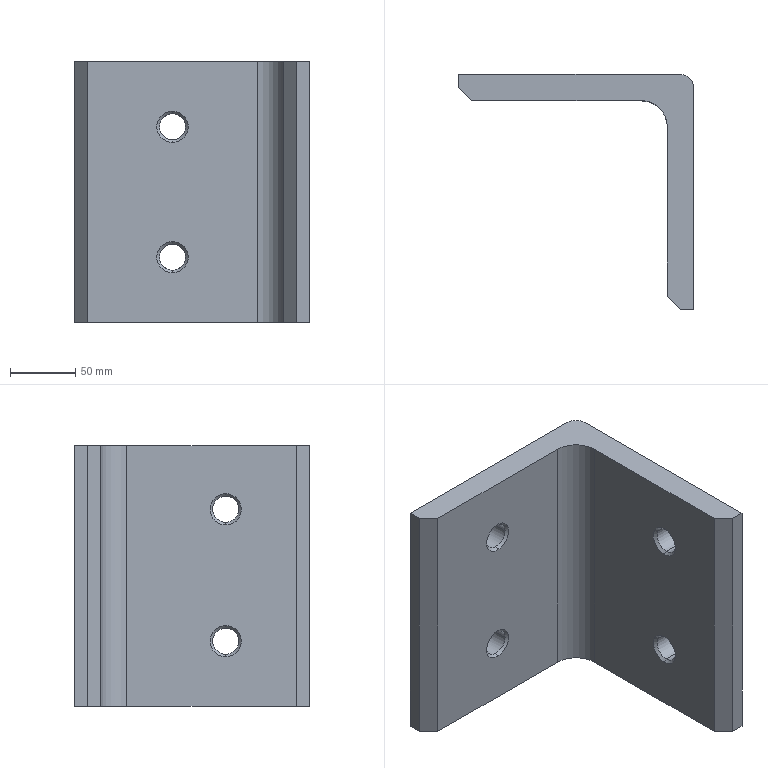Component | SolidWorks | U-shapedPlate-1 | 1 solid | 28 faces | box 180 x 180 x 200 mm | volume 1327207 mm3 | cylinder 10 | plane 10 | cone 8 | commonest cylinder face diameters 20 x9 40 x1
build123d program:
from build123d import *

# Parameters (mm, degrees)
BOSS_EXTRUDE1_DEPTH = 100
FILLET1_R           = 10
SKETCH2_R           = 10
CUT_EXTRUDE1_DEPTH  = 473.323
CHAMFER1_SIZE       = 2
SKETCH3_R           = 10
CUT_EXTRUDE2_DEPTH  = 2195.128
CHAMFER2_SIZE       = 2


with BuildPart() as part:
    # Sketch1 → Boss-Extrude1 (new, symmetric)
    with BuildSketch(Plane.XY):
        with BuildLine():
            Line((2186, -433), (2186, -253))
            Line((2186, -253), (2006, -253))
            Line((2006, -253), (2006, -263))
            Line((2006, -263), (2016, -273))
            Line((2016, -273), (2146, -273))
            ThreePointArc((2146, -273), (2160.142, -278.858), (2166, -293))
            Line((2166, -293), (2166, -423))
            Line((2166, -423), (2176, -433))
            Line((2176, -433), (2186, -433))
        make_face()
    extrude(amount=BOSS_EXTRUDE1_DEPTH, both=True)

    # Fillet1
    fillet1_edges = [part.edges().sort_by_distance(p)[0] for p in [
        (2186, -253, 0),
    ]]
    fillet(fillet1_edges, radius=FILLET1_R)

    # Sketch2 → Cut-Extrude1 (cut, through all)
    with BuildSketch(Plane.ZY.offset(-2166)):
        with Locations((-50, -368.825)):
            Circle(SKETCH2_R)
        with Locations((51.119, -368.825)):
            Circle(SKETCH2_R)
    extrude(amount=-CUT_EXTRUDE1_DEPTH, mode=Mode.SUBTRACT)

    # Chamfer1
    chamfer1_edges = [part.edges().sort_by_distance(p)[0] for p in [
        (2166, -368.825, -60),
        (2166, -368.825, 41.119),
    ]]
    chamfer(chamfer1_edges, length=CHAMFER1_SIZE)

    # Sketch3 → Cut-Extrude2 (cut, through all)
    with BuildSketch(Plane.XZ.offset(273)):
        with Locations((2081.035, 50)):
            Circle(SKETCH3_R)
        with Locations(Location((2081.035, -50, 0), (0, 0, 180))):
            Circle(SKETCH3_R)
    extrude(amount=-CUT_EXTRUDE2_DEPTH, mode=Mode.SUBTRACT)

    # Chamfer2
    chamfer2_edges = [part.edges().sort_by_distance(p)[0] for p in [
        (2071.035, -273, 50),
        (2091.035, -273, -50),
    ]]
    chamfer(chamfer2_edges, length=CHAMFER2_SIZE)


solid = part.part

# Placed as in the assembly
solid = solid.moved(Location((0, 0, -255), (0, 0, 0)))
STEP:
#1=COLOUR_RGB('',0.7922,0.8196,0.9333);
#2=FILL_AREA_STYLE_COLOUR('',#1);
#3=FILL_AREA_STYLE('',(#2));
#4=SURFACE_STYLE_FILL_AREA(#3);
#5=SURFACE_SIDE_STYLE('',(#4));
#6=SURFACE_STYLE_USAGE(.BOTH.,#5);
#7=PRESENTATION_STYLE_ASSIGNMENT((#6));
#8=CARTESIAN_POINT('',(81.931,-10.669,-7.677));
#9=VERTEX_POINT('',#8);
#10=CARTESIAN_POINT('',(81.537,-10.669,-8.071));
#11=VERTEX_POINT('',#10);
#12=CARTESIAN_POINT('',(81.931,-10.669,-8.071));
#13=DIRECTION('',(0.,-1.,0.));
#14=DIRECTION('',(0.,0.,1.));
#15=AXIS2_PLACEMENT_3D('',#12,#13,#14);
#16=CIRCLE('',#15,0.3937);
#17=EDGE_CURVE('',#9,#11,#16,.T.);
#18=ORIENTED_EDGE('',*,*,#17,.F.);
#19=CARTESIAN_POINT('',(81.931,-10.748,-7.598));
#20=VERTEX_POINT('',#19);
#21=CARTESIAN_POINT('',(81.931,-10.669,-7.677));
#22=DIRECTION('',(0.,-0.7071,0.7071));
#23=VECTOR('',#22,39.37);
#24=LINE('',#21,#23);
#25=EDGE_CURVE('',#9,#20,#24,.T.);
#26=ORIENTED_EDGE('',*,*,#25,.T.);
#27=CARTESIAN_POINT('',(81.931,-10.748,-8.543));
#28=VERTEX_POINT('',#27);
#29=CARTESIAN_POINT('',(81.931,-10.748,-8.071));
#30=DIRECTION('',(-0.,1.,0.));
#31=DIRECTION('',(-1.,0.,0.));
#32=AXIS2_PLACEMENT_3D('',#29,#30,#31);
#33=CIRCLE('',#32,0.4724);
#34=EDGE_CURVE('',#28,#20,#33,.T.);
#35=ORIENTED_EDGE('',*,*,#34,.F.);
#36=CARTESIAN_POINT('',(81.931,-10.669,-8.465));
#37=VERTEX_POINT('',#36);
#38=CARTESIAN_POINT('',(81.931,-10.669,-8.465));
#39=DIRECTION('',(0.,-0.7071,-0.7071));
#40=VECTOR('',#39,39.37);
#41=LINE('',#38,#40);
#42=EDGE_CURVE('',#37,#28,#41,.T.);
#43=ORIENTED_EDGE('',*,*,#42,.F.);
#44=CARTESIAN_POINT('',(81.931,-10.669,-8.071));
#45=DIRECTION('',(0.,-1.,0.));
#46=DIRECTION('',(0.,0.,1.));
#47=AXIS2_PLACEMENT_3D('',#44,#45,#46);
#48=CIRCLE('',#47,0.3937);
#49=EDGE_CURVE('',#11,#37,#48,.T.);
#50=ORIENTED_EDGE('',*,*,#49,.F.);
#51=EDGE_LOOP('',(#18,#26,#35,#43,#50));
#52=FACE_OUTER_BOUND('',#51,.T.);
#53=CARTESIAN_POINT('',(81.931,-10.669,-8.071));
#54=DIRECTION('',(0.,-1.,0.));
#55=DIRECTION('',(0.,0.,-1.));
#56=AXIS2_PLACEMENT_3D('',#53,#54,#55);
#57=CONICAL_SURFACE('',#56,0.3937,0.7854);
#58=ADVANCED_FACE('',(#52),#57,.F.);
#59=CARTESIAN_POINT('',(81.931,-10.669,-11.614));
#60=VERTEX_POINT('',#59);
#61=CARTESIAN_POINT('',(81.537,-10.669,-12.008));
#62=VERTEX_POINT('',#61);
#63=CARTESIAN_POINT('',(81.931,-10.669,-12.008));
#64=DIRECTION('',(0.,-1.,0.));
#65=DIRECTION('',(0.,0.,1.));
#66=AXIS2_PLACEMENT_3D('',#63,#64,#65);
#67=CIRCLE('',#66,0.3937);
#68=EDGE_CURVE('',#60,#62,#67,.T.);
#69=ORIENTED_EDGE('',*,*,#68,.F.);
#70=CARTESIAN_POINT('',(81.931,-10.748,-11.535));
#71=VERTEX_POINT('',#70);
#72=CARTESIAN_POINT('',(81.931,-10.669,-11.614));
#73=DIRECTION('',(0.,-0.7071,0.7071));
#74=VECTOR('',#73,39.37);
#75=LINE('',#72,#74);
#76=EDGE_CURVE('',#60,#71,#75,.T.);
#77=ORIENTED_EDGE('',*,*,#76,.T.);
#78=CARTESIAN_POINT('',(81.931,-10.748,-12.48));
#79=VERTEX_POINT('',#78);
#80=CARTESIAN_POINT('',(81.931,-10.748,-12.008));
#81=DIRECTION('',(-0.,1.,0.));
#82=DIRECTION('',(-1.,0.,0.));
#83=AXIS2_PLACEMENT_3D('',#80,#81,#82);
#84=CIRCLE('',#83,0.4724);
#85=EDGE_CURVE('',#79,#71,#84,.T.);
#86=ORIENTED_EDGE('',*,*,#85,.F.);
#87=CARTESIAN_POINT('',(81.931,-10.669,-12.402));
#88=VERTEX_POINT('',#87);
#89=CARTESIAN_POINT('',(81.931,-10.669,-12.402));
#90=DIRECTION('',(0.,-0.7071,-0.7071));
#91=VECTOR('',#90,39.37);
#92=LINE('',#89,#91);
#93=EDGE_CURVE('',#88,#79,#92,.T.);
#94=ORIENTED_EDGE('',*,*,#93,.F.);
#95=CARTESIAN_POINT('',(81.931,-10.669,-12.008));
#96=DIRECTION('',(0.,-1.,0.));
#97=DIRECTION('',(0.,0.,1.));
#98=AXIS2_PLACEMENT_3D('',#95,#96,#97);
#99=CIRCLE('',#98,0.3937);
#100=EDGE_CURVE('',#62,#88,#99,.T.);
#101=ORIENTED_EDGE('',*,*,#100,.F.);
#102=EDGE_LOOP('',(#69,#77,#86,#94,#101));
#103=FACE_OUTER_BOUND('',#102,.T.);
#104=CARTESIAN_POINT('',(81.931,-10.669,-12.008));
#105=DIRECTION('',(0.,-1.,0.));
#106=DIRECTION('',(0.,0.,-1.));
#107=AXIS2_PLACEMENT_3D('',#104,#105,#106);
#108=CONICAL_SURFACE('',#107,0.3937,0.7854);
#109=ADVANCED_FACE('',(#103),#108,.F.);
#110=CARTESIAN_POINT('',(81.537,-9.961,-8.071));
#111=VERTEX_POINT('',#110);
#112=CARTESIAN_POINT('',(82.324,-9.961,-8.071));
#113=VERTEX_POINT('',#112);
#114=CARTESIAN_POINT('',(81.931,-9.961,-8.071));
#115=DIRECTION('',(0.,-1.,0.));
#116=DIRECTION('',(1.,0.,0.));
#117=AXIS2_PLACEMENT_3D('',#114,#115,#116);
#118=CIRCLE('',#117,0.3937);
#119=EDGE_CURVE('',#111,#113,#118,.T.);
#120=ORIENTED_EDGE('',*,*,#119,.F.);
#121=CARTESIAN_POINT('',(81.537,-9.961,-8.071));
#122=DIRECTION('',(0.,-1.,0.));
#123=VECTOR('',#122,39.37);
#124=LINE('',#121,#123);
#125=EDGE_CURVE('',#111,#11,#124,.T.);
#126=ORIENTED_EDGE('',*,*,#125,.T.);
#127=ORIENTED_EDGE('',*,*,#49,.T.);
#128=CARTESIAN_POINT('',(82.324,-10.669,-8.071));
#129=VERTEX_POINT('',#128);
#130=CARTESIAN_POINT('',(81.931,-10.669,-8.071));
#131=DIRECTION('',(0.,-1.,0.));
#132=DIRECTION('',(0.,0.,1.));
#133=AXIS2_PLACEMENT_3D('',#130,#131,#132);
#134=CIRCLE('',#133,0.3937);
#135=EDGE_CURVE('',#37,#129,#134,.T.);
#136=ORIENTED_EDGE('',*,*,#135,.T.);
#137=CARTESIAN_POINT('',(82.324,-9.961,-8.071));
#138=DIRECTION('',(0.,-1.,0.));
#139=VECTOR('',#138,39.37);
#140=LINE('',#137,#139);
#141=EDGE_CURVE('',#113,#129,#140,.T.);
#142=ORIENTED_EDGE('',*,*,#141,.F.);
#143=EDGE_LOOP('',(#120,#126,#127,#136,#142));
#144=FACE_OUTER_BOUND('',#143,.T.);
#145=CARTESIAN_POINT('',(81.931,-9.961,-8.071));
#146=DIRECTION('',(0.,-1.,0.));
#147=DIRECTION('',(1.,0.,0.));
#148=AXIS2_PLACEMENT_3D('',#145,#146,#147);
#149=CYLINDRICAL_SURFACE('',#148,0.3937);
#150=ADVANCED_FACE('',(#144),#149,.F.);
#151=CARTESIAN_POINT('',(81.537,-9.961,-12.008));
#152=VERTEX_POINT('',#151);
#153=CARTESIAN_POINT('',(82.324,-9.961,-12.008));
#154=VERTEX_POINT('',#153);
#155=CARTESIAN_POINT('',(81.931,-9.961,-12.008));
#156=DIRECTION('',(0.,-1.,0.));
#157=DIRECTION('',(-1.,0.,0.));
#158=AXIS2_PLACEMENT_3D('',#155,#156,#157);
#159=CIRCLE('',#158,0.3937);
#160=EDGE_CURVE('',#152,#154,#159,.T.);
#161=ORIENTED_EDGE('',*,*,#160,.F.);
#162=CARTESIAN_POINT('',(81.537,-9.961,-12.008));
#163=DIRECTION('',(0.,-1.,0.));
#164=VECTOR('',#163,39.37);
#165=LINE('',#162,#164);
#166=EDGE_CURVE('',#152,#62,#165,.T.);
#167=ORIENTED_EDGE('',*,*,#166,.T.);
#168=ORIENTED_EDGE('',*,*,#100,.T.);
#169=CARTESIAN_POINT('',(82.324,-10.669,-12.008));
#170=VERTEX_POINT('',#169);
#171=CARTESIAN_POINT('',(81.931,-10.669,-12.008));
#172=DIRECTION('',(0.,-1.,0.));
#173=DIRECTION('',(0.,0.,1.));
#174=AXIS2_PLACEMENT_3D('',#171,#172,#173);
#175=CIRCLE('',#174,0.3937);
#176=EDGE_CURVE('',#88,#170,#175,.T.);
#177=ORIENTED_EDGE('',*,*,#176,.T.);
#178=CARTESIAN_POINT('',(82.324,-9.961,-12.008));
#179=DIRECTION('',(0.,-1.,0.));
#180=VECTOR('',#179,39.37);
#181=LINE('',#178,#180);
#182=EDGE_CURVE('',#154,#170,#181,.T.);
#183=ORIENTED_EDGE('',*,*,#182,.F.);
#184=EDGE_LOOP('',(#161,#167,#168,#177,#183));
#185=FACE_OUTER_BOUND('',#184,.T.);
#186=CARTESIAN_POINT('',(81.931,-9.961,-12.008));
#187=DIRECTION('',(0.,-1.,0.));
#188=DIRECTION('',(1.,0.,0.));
#189=AXIS2_PLACEMENT_3D('',#186,#187,#188);
#190=CYLINDRICAL_SURFACE('',#189,0.3937);
#191=ADVANCED_FACE('',(#185),#190,.F.);
#192=CARTESIAN_POINT('',(85.354,-14.521,-12.402));
#193=VERTEX_POINT('',#192);
#194=CARTESIAN_POINT('',(85.354,-14.521,-11.614));
#195=VERTEX_POINT('',#194);
#196=CARTESIAN_POINT('',(85.354,-14.521,-12.008));
#197=DIRECTION('',(-1.,0.,0.));
#198=DIRECTION('',(0.,0.,-1.));
#199=AXIS2_PLACEMENT_3D('',#196,#197,#198);
#200=CIRCLE('',#199,0.3937);
#201=EDGE_CURVE('',#193,#195,#200,.T.);
#202=ORIENTED_EDGE('',*,*,#201,.F.);
#203=CARTESIAN_POINT('',(85.276,-14.521,-12.48));
#204=VERTEX_POINT('',#203);
#205=CARTESIAN_POINT('',(85.354,-14.521,-12.402));
#206=DIRECTION('',(-0.7071,0.,-0.7071));
#207=VECTOR('',#206,39.37);
#208=LINE('',#205,#207);
#209=EDGE_CURVE('',#193,#204,#208,.T.);
#210=ORIENTED_EDGE('',*,*,#209,.T.);
#211=CARTESIAN_POINT('',(85.276,-14.521,-11.535));
#212=VERTEX_POINT('',#211);
#213=CARTESIAN_POINT('',(85.276,-14.521,-12.008));
#214=DIRECTION('',(1.,0.,0.));
#215=DIRECTION('',(0.,0.,-1.));
#216=AXIS2_PLACEMENT_3D('',#213,#214,#215);
#217=CIRCLE('',#216,0.4724);
#218=EDGE_CURVE('',#212,#204,#217,.T.);
#219=ORIENTED_EDGE('',*,*,#218,.F.);
#220=CARTESIAN_POINT('',(85.354,-14.521,-11.614));
#221=DIRECTION('',(-0.7071,0.,0.7071));
#222=VECTOR('',#221,39.37);
#223=LINE('',#220,#222);
#224=EDGE_CURVE('',#195,#212,#223,.T.);
#225=ORIENTED_EDGE('',*,*,#224,.F.);
#226=EDGE_LOOP('',(#202,#210,#219,#225));
#227=FACE_OUTER_BOUND('',#226,.T.);
#228=CARTESIAN_POINT('',(85.354,-14.521,-12.008));
#229=DIRECTION('',(-1.,0.,0.));
#230=DIRECTION('',(0.,0.,1.));
#231=AXIS2_PLACEMENT_3D('',#228,#229,#230);
#232=CONICAL_SURFACE('',#231,0.3937,0.7854);
#233=ADVANCED_FACE('',(#227),#232,.F.);
#234=CARTESIAN_POINT('',(85.354,-14.521,-8.421));
#235=VERTEX_POINT('',#234);
#236=CARTESIAN_POINT('',(85.354,-14.521,-7.633));
#237=VERTEX_POINT('',#236);
#238=CARTESIAN_POINT('',(85.354,-14.521,-8.027));
#239=DIRECTION('',(-1.,0.,0.));
#240=DIRECTION('',(0.,0.,-1.));
#241=AXIS2_PLACEMENT_3D('',#238,#239,#240);
#242=CIRCLE('',#241,0.3937);
#243=EDGE_CURVE('',#235,#237,#242,.T.);
#244=ORIENTED_EDGE('',*,*,#243,.F.);
#245=CARTESIAN_POINT('',(85.276,-14.521,-8.499));
#246=VERTEX_POINT('',#245);
#247=CARTESIAN_POINT('',(85.354,-14.521,-8.421));
#248=DIRECTION('',(-0.7071,0.,-0.7071));
#249=VECTOR('',#248,39.37);
#250=LINE('',#247,#249);
#251=EDGE_CURVE('',#235,#246,#250,.T.);
#252=ORIENTED_EDGE('',*,*,#251,.T.);
#253=CARTESIAN_POINT('',(85.276,-14.521,-7.554));
#254=VERTEX_POINT('',#253);
#255=CARTESIAN_POINT('',(85.276,-14.521,-8.027));
#256=DIRECTION('',(1.,0.,0.));
#257=DIRECTION('',(0.,0.,-1.));
#258=AXIS2_PLACEMENT_3D('',#255,#256,#257);
#259=CIRCLE('',#258,0.4724);
#260=EDGE_CURVE('',#254,#246,#259,.T.);
#261=ORIENTED_EDGE('',*,*,#260,.F.);
#262=CARTESIAN_POINT('',(85.354,-14.521,-7.633));
#263=DIRECTION('',(-0.7071,0.,0.7071));
#264=VECTOR('',#263,39.37);
#265=LINE('',#262,#264);
#266=EDGE_CURVE('',#237,#254,#265,.T.);
#267=ORIENTED_EDGE('',*,*,#266,.F.);
#268=EDGE_LOOP('',(#244,#252,#261,#267));
#269=FACE_OUTER_BOUND('',#268,.T.);
#270=CARTESIAN_POINT('',(85.354,-14.521,-8.027));
#271=DIRECTION('',(-1.,0.,0.));
#272=DIRECTION('',(0.,0.,1.));
#273=AXIS2_PLACEMENT_3D('',#270,#271,#272);
#274=CONICAL_SURFACE('',#273,0.3937,0.7854);
#275=ADVANCED_FACE('',(#269),#274,.F.);
#276=CARTESIAN_POINT('',(86.063,-14.521,-12.402));
#277=VERTEX_POINT('',#276);
#278=CARTESIAN_POINT('',(86.063,-14.521,-11.614));
#279=VERTEX_POINT('',#278);
#280=CARTESIAN_POINT('',(86.063,-14.521,-12.008));
#281=DIRECTION('',(-1.,0.,0.));
#282=DIRECTION('',(0.,0.,1.));
#283=AXIS2_PLACEMENT_3D('',#280,#281,#282);
#284=CIRCLE('',#283,0.3937);
#285=EDGE_CURVE('',#277,#279,#284,.T.);
#286=ORIENTED_EDGE('',*,*,#285,.F.);
#287=CARTESIAN_POINT('',(86.063,-14.521,-12.402));
#288=DIRECTION('',(-1.,0.,0.));
#289=VECTOR('',#288,39.37);
#290=LINE('',#287,#289);
#291=EDGE_CURVE('',#277,#193,#290,.T.);
#292=ORIENTED_EDGE('',*,*,#291,.T.);
#293=ORIENTED_EDGE('',*,*,#201,.T.);
#294=CARTESIAN_POINT('',(86.063,-14.521,-11.614));
#295=DIRECTION('',(-1.,0.,0.));
#296=VECTOR('',#295,39.37);
#297=LINE('',#294,#296);
#298=EDGE_CURVE('',#279,#195,#297,.T.);
#299=ORIENTED_EDGE('',*,*,#298,.F.);
#300=EDGE_LOOP('',(#286,#292,#293,#299));
#301=FACE_OUTER_BOUND('',#300,.T.);
#302=CARTESIAN_POINT('',(86.063,-14.521,-12.008));
#303=DIRECTION('',(-1.,0.,0.));
#304=DIRECTION('',(0.,0.,1.));
#305=AXIS2_PLACEMENT_3D('',#302,#303,#304);
#306=CYLINDRICAL_SURFACE('',#305,0.3937);
#307=ADVANCED_FACE('',(#301),#306,.F.);
#308=CARTESIAN_POINT('',(86.063,-14.521,-8.421));
#309=VERTEX_POINT('',#308);
#310=CARTESIAN_POINT('',(86.063,-14.521,-7.633));
#311=VERTEX_POINT('',#310);
#312=CARTESIAN_POINT('',(86.063,-14.521,-8.027));
#313=DIRECTION('',(-1.,0.,0.));
#314=DIRECTION('',(0.,0.,1.));
#315=AXIS2_PLACEMENT_3D('',#312,#313,#314);
#316=CIRCLE('',#315,0.3937);
#317=EDGE_CURVE('',#309,#311,#316,.T.);
#318=ORIENTED_EDGE('',*,*,#317,.F.);
#319=CARTESIAN_POINT('',(86.063,-14.521,-8.421));
#320=DIRECTION('',(-1.,0.,0.));
#321=VECTOR('',#320,39.37);
#322=LINE('',#319,#321);
#323=EDGE_CURVE('',#309,#235,#322,.T.);
#324=ORIENTED_EDGE('',*,*,#323,.T.);
#325=ORIENTED_EDGE('',*,*,#243,.T.);
#326=CARTESIAN_POINT('',(86.063,-14.521,-7.633));
#327=DIRECTION('',(-1.,0.,0.));
#328=VECTOR('',#327,39.37);
#329=LINE('',#326,#328);
#330=EDGE_CURVE('',#311,#237,#329,.T.);
#331=ORIENTED_EDGE('',*,*,#330,.F.);
#332=EDGE_LOOP('',(#318,#324,#325,#331));
#333=FACE_OUTER_BOUND('',#332,.T.);
#334=CARTESIAN_POINT('',(86.063,-14.521,-8.027));
#335=DIRECTION('',(-1.,0.,0.));
#336=DIRECTION('',(0.,0.,1.));
#337=AXIS2_PLACEMENT_3D('',#334,#335,#336);
#338=CYLINDRICAL_SURFACE('',#337,0.3937);
#339=ADVANCED_FACE('',(#333),#338,.F.);
#340=CARTESIAN_POINT('',(85.669,-17.047,-13.976));
#341=VERTEX_POINT('',#340);
#342=CARTESIAN_POINT('',(86.063,-17.047,-13.976));
#343=VERTEX_POINT('',#342);
#344=CARTESIAN_POINT('',(86.063,-17.047,-13.976));
#345=DIRECTION('',(1.,0.,0.));
#346=VECTOR('',#345,39.37);
#347=LINE('',#344,#346);
#348=EDGE_CURVE('',#341,#343,#347,.T.);
#349=ORIENTED_EDGE('',*,*,#348,.T.);
#350=CARTESIAN_POINT('',(86.063,-17.047,-6.102));
#351=VERTEX_POINT('',#350);
#352=CARTESIAN_POINT('',(86.063,-17.047,-6.102));
#353=DIRECTION('',(0.,0.,-1.));
#354=VECTOR('',#353,39.37);
#355=LINE('',#352,#354);
#356=EDGE_CURVE('',#351,#343,#355,.T.);
#357=ORIENTED_EDGE('',*,*,#356,.F.);
#358=CARTESIAN_POINT('',(85.669,-17.047,-6.102));
#359=VERTEX_POINT('',#358);
#360=CARTESIAN_POINT('',(86.063,-17.047,-6.102));
#361=DIRECTION('',(1.,0.,0.));
#362=VECTOR('',#361,39.37);
#363=LINE('',#360,#362);
#364=EDGE_CURVE('',#359,#351,#363,.T.);
#365=ORIENTED_EDGE('',*,*,#364,.F.);
#366=CARTESIAN_POINT('',(85.669,-17.047,-6.102));
#367=DIRECTION('',(0.,0.,-1.));
#368=VECTOR('',#367,39.37);
#369=LINE('',#366,#368);
#370=EDGE_CURVE('',#359,#341,#369,.T.);
#371=ORIENTED_EDGE('',*,*,#370,.T.);
#372=EDGE_LOOP('',(#349,#357,#365,#371));
#373=FACE_OUTER_BOUND('',#372,.T.);
#374=CARTESIAN_POINT('',(86.063,-17.047,-6.102));
#375=DIRECTION('',(0.,1.,0.));
#376=DIRECTION('',(0.,0.,1.));
#377=AXIS2_PLACEMENT_3D('',#374,#375,#376);
#378=PLANE('',#377);
#379=ADVANCED_FACE('',(#373),#378,.F.);
#380=CARTESIAN_POINT('',(86.063,-14.521,-12.008));
#381=DIRECTION('',(-1.,0.,0.));
#382=DIRECTION('',(0.,0.,1.));
#383=AXIS2_PLACEMENT_3D('',#380,#381,#382);
#384=CIRCLE('',#383,0.3937);
#385=EDGE_CURVE('',#279,#277,#384,.T.);
#386=ORIENTED_EDGE('',*,*,#385,.T.);
#387=ORIENTED_EDGE('',*,*,#285,.T.);
#388=EDGE_LOOP('',(#386,#387));
#389=FACE_BOUND('',#388,.T.);
#390=CARTESIAN_POINT('',(86.063,-14.521,-8.027));
#391=DIRECTION('',(-1.,0.,0.));
#392=DIRECTION('',(0.,0.,1.));
#393=AXIS2_PLACEMENT_3D('',#390,#391,#392);
#394=CIRCLE('',#393,0.3937);
#395=EDGE_CURVE('',#311,#309,#394,.T.);
#396=ORIENTED_EDGE('',*,*,#395,.T.);
#397=ORIENTED_EDGE('',*,*,#317,.T.);
#398=EDGE_LOOP('',(#396,#397));
#399=FACE_BOUND('',#398,.T.);
#400=CARTESIAN_POINT('',(86.063,-10.354,-13.976));
#401=VERTEX_POINT('',#400);
#402=CARTESIAN_POINT('',(86.063,-17.047,-13.976));
#403=DIRECTION('',(0.,1.,0.));
#404=VECTOR('',#403,39.37);
#405=LINE('',#402,#404);
#406=EDGE_CURVE('',#343,#401,#405,.T.);
#407=ORIENTED_EDGE('',*,*,#406,.T.);
#408=CARTESIAN_POINT('',(86.063,-10.354,-6.102));
#409=VERTEX_POINT('',#408);
#410=CARTESIAN_POINT('',(86.063,-10.354,-6.102));
#411=DIRECTION('',(0.,0.,1.));
#412=VECTOR('',#411,39.37);
#413=LINE('',#410,#412);
#414=EDGE_CURVE('',#401,#409,#413,.T.);
#415=ORIENTED_EDGE('',*,*,#414,.T.);
#416=CARTESIAN_POINT('',(86.063,-17.047,-6.102));
#417=DIRECTION('',(0.,1.,0.));
#418=VECTOR('',#417,39.37);
#419=LINE('',#416,#418);
#420=EDGE_CURVE('',#351,#409,#419,.T.);
#421=ORIENTED_EDGE('',*,*,#420,.F.);
#422=ORIENTED_EDGE('',*,*,#356,.T.);
#423=EDGE_LOOP('',(#407,#415,#421,#422));
#424=FACE_OUTER_BOUND('',#423,.T.);
#425=CARTESIAN_POINT('',(86.063,-17.047,-6.102));
#426=DIRECTION('',(-1.,0.,0.));
#427=DIRECTION('',(-0.,-1.,0.));
#428=AXIS2_PLACEMENT_3D('',#425,#426,#427);
#429=PLANE('',#428);
#430=ADVANCED_FACE('',(#389,#399,#424),#429,.F.);
#431=CARTESIAN_POINT('',(81.931,-9.961,-8.071));
#432=DIRECTION('',(0.,-1.,0.));
#433=DIRECTION('',(1.,0.,0.));
#434=AXIS2_PLACEMENT_3D('',#431,#432,#433);
#435=CIRCLE('',#434,0.3937);
#436=EDGE_CURVE('',#113,#111,#435,.T.);
#437=ORIENTED_EDGE('',*,*,#436,.T.);
#438=ORIENTED_EDGE('',*,*,#119,.T.);
#439=EDGE_LOOP('',(#437,#438));
#440=FACE_BOUND('',#439,.T.);
#441=CARTESIAN_POINT('',(81.931,-9.961,-12.008));
#442=DIRECTION('',(0.,-1.,0.));
#443=DIRECTION('',(-1.,0.,0.));
#444=AXIS2_PLACEMENT_3D('',#441,#442,#443);
#445=CIRCLE('',#444,0.3937);
#446=EDGE_CURVE('',#154,#152,#445,.T.);
#447=ORIENTED_EDGE('',*,*,#446,.T.);
#448=ORIENTED_EDGE('',*,*,#160,.T.);
#449=EDGE_LOOP('',(#447,#448));
#450=FACE_BOUND('',#449,.T.);
#451=CARTESIAN_POINT('',(85.669,-9.961,-6.102));
#452=VERTEX_POINT('',#451);
#453=CARTESIAN_POINT('',(78.976,-9.961,-6.102));
#454=VERTEX_POINT('',#453);
#455=CARTESIAN_POINT('',(86.063,-9.961,-6.102));
#456=DIRECTION('',(-1.,0.,0.));
#457=VECTOR('',#456,39.37);
#458=LINE('',#455,#457);
#459=EDGE_CURVE('',#452,#454,#458,.T.);
#460=ORIENTED_EDGE('',*,*,#459,.F.);
#461=CARTESIAN_POINT('',(85.669,-9.961,-13.976));
#462=VERTEX_POINT('',#461);
#463=CARTESIAN_POINT('',(85.669,-9.961,-6.102));
#464=DIRECTION('',(0.,0.,-1.));
#465=VECTOR('',#464,39.37);
#466=LINE('',#463,#465);
#467=EDGE_CURVE('',#452,#462,#466,.T.);
#468=ORIENTED_EDGE('',*,*,#467,.T.);
#469=CARTESIAN_POINT('',(78.976,-9.961,-13.976));
#470=VERTEX_POINT('',#469);
#471=CARTESIAN_POINT('',(86.063,-9.961,-13.976));
#472=DIRECTION('',(-1.,0.,0.));
#473=VECTOR('',#472,39.37);
#474=LINE('',#471,#473);
#475=EDGE_CURVE('',#462,#470,#474,.T.);
#476=ORIENTED_EDGE('',*,*,#475,.T.);
#477=CARTESIAN_POINT('',(78.976,-9.961,-6.102));
#478=DIRECTION('',(0.,0.,-1.));
#479=VECTOR('',#478,39.37);
#480=LINE('',#477,#479);
#481=EDGE_CURVE('',#454,#470,#480,.T.);
#482=ORIENTED_EDGE('',*,*,#481,.F.);
#483=EDGE_LOOP('',(#460,#468,#476,#482));
#484=FACE_OUTER_BOUND('',#483,.T.);
#485=CARTESIAN_POINT('',(86.063,-9.961,-6.102));
#486=DIRECTION('',(0.,-1.,0.));
#487=DIRECTION('',(0.,0.,-1.));
#488=AXIS2_PLACEMENT_3D('',#485,#486,#487);
#489=PLANE('',#488);
#490=ADVANCED_FACE('',(#440,#450,#484),#489,.F.);
#491=CARTESIAN_POINT('',(78.976,-10.354,-13.976));
#492=VERTEX_POINT('',#491);
#493=CARTESIAN_POINT('',(78.976,-10.354,-13.976));
#494=DIRECTION('',(0.,-1.,0.));
#495=VECTOR('',#494,39.37);
#496=LINE('',#493,#495);
#497=EDGE_CURVE('',#470,#492,#496,.T.);
#498=ORIENTED_EDGE('',*,*,#497,.T.);
#499=CARTESIAN_POINT('',(78.976,-10.354,-6.102));
#500=VERTEX_POINT('',#499);
#501=CARTESIAN_POINT('',(78.976,-10.354,-6.102));
#502=DIRECTION('',(0.,0.,-1.));
#503=VECTOR('',#502,39.37);
#504=LINE('',#501,#503);
#505=EDGE_CURVE('',#500,#492,#504,.T.);
#506=ORIENTED_EDGE('',*,*,#505,.F.);
#507=CARTESIAN_POINT('',(78.976,-10.354,-6.102));
#508=DIRECTION('',(0.,-1.,0.));
#509=VECTOR('',#508,39.37);
#510=LINE('',#507,#509);
#511=EDGE_CURVE('',#454,#500,#510,.T.);
#512=ORIENTED_EDGE('',*,*,#511,.F.);
#513=ORIENTED_EDGE('',*,*,#481,.T.);
#514=EDGE_LOOP('',(#498,#506,#512,#513));
#515=FACE_OUTER_BOUND('',#514,.T.);
#516=CARTESIAN_POINT('',(78.976,-10.354,-6.102));
#517=DIRECTION('',(1.,0.,0.));
#518=DIRECTION('',(0.,0.,-1.));
#519=AXIS2_PLACEMENT_3D('',#516,#517,#518);
#520=PLANE('',#519);
#521=ADVANCED_FACE('',(#515),#520,.F.);
#522=CARTESIAN_POINT('',(79.37,-10.748,-13.976));
#523=VERTEX_POINT('',#522);
#524=CARTESIAN_POINT('',(79.37,-10.748,-13.976));
#525=DIRECTION('',(0.7071,-0.7071,0.));
#526=VECTOR('',#525,39.37);
#527=LINE('',#524,#526);
#528=EDGE_CURVE('',#492,#523,#527,.T.);
#529=ORIENTED_EDGE('',*,*,#528,.T.);
#530=CARTESIAN_POINT('',(79.37,-10.748,-6.102));
#531=VERTEX_POINT('',#530);
#532=CARTESIAN_POINT('',(79.37,-10.748,-6.102));
#533=DIRECTION('',(0.,0.,-1.));
#534=VECTOR('',#533,39.37);
#535=LINE('',#532,#534);
#536=EDGE_CURVE('',#531,#523,#535,.T.);
#537=ORIENTED_EDGE('',*,*,#536,.F.);
#538=CARTESIAN_POINT('',(79.37,-10.748,-6.102));
#539=DIRECTION('',(0.7071,-0.7071,0.));
#540=VECTOR('',#539,39.37);
#541=LINE('',#538,#540);
#542=EDGE_CURVE('',#500,#531,#541,.T.);
#543=ORIENTED_EDGE('',*,*,#542,.F.);
#544=ORIENTED_EDGE('',*,*,#505,.T.);
#545=EDGE_LOOP('',(#529,#537,#543,#544));
#546=FACE_OUTER_BOUND('',#545,.T.);
#547=CARTESIAN_POINT('',(79.37,-10.748,-6.102));
#548=DIRECTION('',(0.7071,0.7071,0.));
#549=DIRECTION('',(-0.7071,0.7071,0.));
#550=AXIS2_PLACEMENT_3D('',#547,#548,#549);
#551=PLANE('',#550);
#552=ADVANCED_FACE('',(#546),#551,.F.);
#553=ORIENTED_EDGE('',*,*,#85,.T.);
#554=CARTESIAN_POINT('',(81.931,-10.748,-12.008));
#555=DIRECTION('',(-0.,1.,0.));
#556=DIRECTION('',(-1.,0.,0.));
#557=AXIS2_PLACEMENT_3D('',#554,#555,#556);
#558=CIRCLE('',#557,0.4724);
#559=EDGE_CURVE('',#71,#79,#558,.T.);
#560=ORIENTED_EDGE('',*,*,#559,.T.);
#561=EDGE_LOOP('',(#553,#560));
#562=FACE_BOUND('',#561,.T.);
#563=ORIENTED_EDGE('',*,*,#34,.T.);
#564=CARTESIAN_POINT('',(81.931,-10.748,-8.071));
#565=DIRECTION('',(-0.,1.,0.));
#566=DIRECTION('',(-1.,0.,0.));
#567=AXIS2_PLACEMENT_3D('',#564,#565,#566);
#568=CIRCLE('',#567,0.4724);
#569=EDGE_CURVE('',#20,#28,#568,.T.);
#570=ORIENTED_EDGE('',*,*,#569,.T.);
#571=EDGE_LOOP('',(#563,#570));
#572=FACE_BOUND('',#571,.T.);
#573=CARTESIAN_POINT('',(84.488,-10.748,-13.976));
#574=VERTEX_POINT('',#573);
#575=CARTESIAN_POINT('',(84.488,-10.748,-13.976));
#576=DIRECTION('',(1.,0.,0.));
#577=VECTOR('',#576,39.37);
#578=LINE('',#575,#577);
#579=EDGE_CURVE('',#523,#574,#578,.T.);
#580=ORIENTED_EDGE('',*,*,#579,.T.);
#581=CARTESIAN_POINT('',(84.488,-10.748,-6.102));
#582=VERTEX_POINT('',#581);
#583=CARTESIAN_POINT('',(84.488,-10.748,-6.102));
#584=DIRECTION('',(0.,0.,-1.));
#585=VECTOR('',#584,39.37);
#586=LINE('',#583,#585);
#587=EDGE_CURVE('',#582,#574,#586,.T.);
#588=ORIENTED_EDGE('',*,*,#587,.F.);
#589=CARTESIAN_POINT('',(84.488,-10.748,-6.102));
#590=DIRECTION('',(1.,0.,0.));
#591=VECTOR('',#590,39.37);
#592=LINE('',#589,#591);
#593=EDGE_CURVE('',#531,#582,#592,.T.);
#594=ORIENTED_EDGE('',*,*,#593,.F.);
#595=ORIENTED_EDGE('',*,*,#536,.T.);
#596=EDGE_LOOP('',(#580,#588,#594,#595));
#597=FACE_OUTER_BOUND('',#596,.T.);
#598=CARTESIAN_POINT('',(84.488,-10.748,-6.102));
#599=DIRECTION('',(-0.,1.,0.));
#600=DIRECTION('',(-1.,-0.,0.));
#601=AXIS2_PLACEMENT_3D('',#598,#599,#600);
#602=PLANE('',#601);
#603=ADVANCED_FACE('',(#562,#572,#597),#602,.F.);
#604=CARTESIAN_POINT('',(85.276,-11.535,-13.976));
#605=VERTEX_POINT('',#604);
#606=CARTESIAN_POINT('',(84.488,-11.535,-13.976));
#607=DIRECTION('',(0.,0.,-1.));
#608=DIRECTION('',(1.,0.,0.));
#609=AXIS2_PLACEMENT_3D('',#606,#607,#608);
#610=CIRCLE('',#609,0.7874);
#611=EDGE_CURVE('',#574,#605,#610,.T.);
#612=ORIENTED_EDGE('',*,*,#611,.T.);
#613=CARTESIAN_POINT('',(85.276,-11.535,-6.102));
#614=VERTEX_POINT('',#613);
#615=CARTESIAN_POINT('',(85.276,-11.535,-6.102));
#616=DIRECTION('',(0.,0.,-1.));
#617=VECTOR('',#616,39.37);
#618=LINE('',#615,#617);
#619=EDGE_CURVE('',#614,#605,#618,.T.);
#620=ORIENTED_EDGE('',*,*,#619,.F.);
#621=CARTESIAN_POINT('',(84.488,-11.535,-6.102));
#622=DIRECTION('',(0.,0.,-1.));
#623=DIRECTION('',(1.,0.,0.));
#624=AXIS2_PLACEMENT_3D('',#621,#622,#623);
#625=CIRCLE('',#624,0.7874);
#626=EDGE_CURVE('',#582,#614,#625,.T.);
#627=ORIENTED_EDGE('',*,*,#626,.F.);
#628=ORIENTED_EDGE('',*,*,#587,.T.);
#629=EDGE_LOOP('',(#612,#620,#627,#628));
#630=FACE_OUTER_BOUND('',#629,.T.);
#631=CARTESIAN_POINT('',(84.488,-11.535,-6.102));
#632=DIRECTION('',(0.,0.,-1.));
#633=DIRECTION('',(-1.,0.,0.));
#634=AXIS2_PLACEMENT_3D('',#631,#632,#633);
#635=CYLINDRICAL_SURFACE('',#634,0.7874);
#636=ADVANCED_FACE('',(#630),#635,.F.);
#637=ORIENTED_EDGE('',*,*,#260,.T.);
#638=CARTESIAN_POINT('',(85.276,-14.521,-8.027));
#639=DIRECTION('',(1.,0.,0.));
#640=DIRECTION('',(0.,0.,-1.));
#641=AXIS2_PLACEMENT_3D('',#638,#639,#640);
#642=CIRCLE('',#641,0.4724);
#643=EDGE_CURVE('',#246,#254,#642,.T.);
#644=ORIENTED_EDGE('',*,*,#643,.T.);
#645=EDGE_LOOP('',(#637,#644));
#646=FACE_BOUND('',#645,.T.);
#647=ORIENTED_EDGE('',*,*,#218,.T.);
#648=CARTESIAN_POINT('',(85.276,-14.521,-12.008));
#649=DIRECTION('',(1.,0.,0.));
#650=DIRECTION('',(0.,0.,-1.));
#651=AXIS2_PLACEMENT_3D('',#648,#649,#650);
#652=CIRCLE('',#651,0.4724);
#653=EDGE_CURVE('',#204,#212,#652,.T.);
#654=ORIENTED_EDGE('',*,*,#653,.T.);
#655=EDGE_LOOP('',(#647,#654));
#656=FACE_BOUND('',#655,.T.);
#657=CARTESIAN_POINT('',(85.276,-16.654,-13.976));
#658=VERTEX_POINT('',#657);
#659=CARTESIAN_POINT('',(85.276,-16.654,-13.976));
#660=DIRECTION('',(0.,-1.,0.));
#661=VECTOR('',#660,39.37);
#662=LINE('',#659,#661);
#663=EDGE_CURVE('',#605,#658,#662,.T.);
#664=ORIENTED_EDGE('',*,*,#663,.T.);
#665=CARTESIAN_POINT('',(85.276,-16.654,-6.102));
#666=VERTEX_POINT('',#665);
#667=CARTESIAN_POINT('',(85.276,-16.654,-6.102));
#668=DIRECTION('',(0.,0.,-1.));
#669=VECTOR('',#668,39.37);
#670=LINE('',#667,#669);
#671=EDGE_CURVE('',#666,#658,#670,.T.);
#672=ORIENTED_EDGE('',*,*,#671,.F.);
#673=CARTESIAN_POINT('',(85.276,-16.654,-6.102));
#674=DIRECTION('',(0.,-1.,0.));
#675=VECTOR('',#674,39.37);
#676=LINE('',#673,#675);
#677=EDGE_CURVE('',#614,#666,#676,.T.);
#678=ORIENTED_EDGE('',*,*,#677,.F.);
#679=ORIENTED_EDGE('',*,*,#619,.T.);
#680=EDGE_LOOP('',(#664,#672,#678,#679));
#681=FACE_OUTER_BOUND('',#680,.T.);
#682=CARTESIAN_POINT('',(85.276,-16.654,-6.102));
#683=DIRECTION('',(1.,0.,0.));
#684=DIRECTION('',(0.,0.,-1.));
#685=AXIS2_PLACEMENT_3D('',#682,#683,#684);
#686=PLANE('',#685);
#687=ADVANCED_FACE('',(#646,#656,#681),#686,.F.);
#688=CARTESIAN_POINT('',(85.669,-17.047,-13.976));
#689=DIRECTION('',(0.7071,-0.7071,0.));
#690=VECTOR('',#689,39.37);
#691=LINE('',#688,#690);
#692=EDGE_CURVE('',#658,#341,#691,.T.);
#693=ORIENTED_EDGE('',*,*,#692,.T.);
#694=ORIENTED_EDGE('',*,*,#370,.F.);
#695=CARTESIAN_POINT('',(85.669,-17.047,-6.102));
#696=DIRECTION('',(0.7071,-0.7071,0.));
#697=VECTOR('',#696,39.37);
#698=LINE('',#695,#697);
#699=EDGE_CURVE('',#666,#359,#698,.T.);
#700=ORIENTED_EDGE('',*,*,#699,.F.);
#701=ORIENTED_EDGE('',*,*,#671,.T.);
#702=EDGE_LOOP('',(#693,#694,#700,#701));
#703=FACE_OUTER_BOUND('',#702,.T.);
#704=CARTESIAN_POINT('',(85.669,-17.047,-6.102));
#705=DIRECTION('',(0.7071,0.7071,0.));
#706=DIRECTION('',(-0.7071,0.7071,0.));
#707=AXIS2_PLACEMENT_3D('',#704,#705,#706);
#708=PLANE('',#707);
#709=ADVANCED_FACE('',(#703),#708,.F.);
#710=ORIENTED_EDGE('',*,*,#420,.T.);
#711=CARTESIAN_POINT('',(85.669,-10.354,-6.102));
#712=DIRECTION('',(0.,0.,1.));
#713=DIRECTION('',(1.,0.,0.));
#714=AXIS2_PLACEMENT_3D('',#711,#712,#713);
#715=CIRCLE('',#714,0.3937);
#716=EDGE_CURVE('',#409,#452,#715,.T.);
#717=ORIENTED_EDGE('',*,*,#716,.T.);
#718=ORIENTED_EDGE('',*,*,#459,.T.);
#719=ORIENTED_EDGE('',*,*,#511,.T.);
#720=ORIENTED_EDGE('',*,*,#542,.T.);
#721=ORIENTED_EDGE('',*,*,#593,.T.);
#722=ORIENTED_EDGE('',*,*,#626,.T.);
#723=ORIENTED_EDGE('',*,*,#677,.T.);
#724=ORIENTED_EDGE('',*,*,#699,.T.);
#725=ORIENTED_EDGE('',*,*,#364,.T.);
#726=EDGE_LOOP('',(#710,#717,#718,#719,#720,#721,#722,#723,#724,#725));
#727=FACE_OUTER_BOUND('',#726,.T.);
#728=CARTESIAN_POINT('',(84.488,-11.535,-6.102));
#729=DIRECTION('',(0.,0.,1.));
#730=DIRECTION('',(1.,0.,0.));
#731=AXIS2_PLACEMENT_3D('',#728,#729,#730);
#732=PLANE('',#731);
#733=ADVANCED_FACE('',(#727),#732,.T.);
#734=ORIENTED_EDGE('',*,*,#475,.F.);
#735=CARTESIAN_POINT('',(85.669,-10.354,-13.976));
#736=DIRECTION('',(0.,0.,-1.));
#737=DIRECTION('',(1.,0.,0.));
#738=AXIS2_PLACEMENT_3D('',#735,#736,#737);
#739=CIRCLE('',#738,0.3937);
#740=EDGE_CURVE('',#462,#401,#739,.T.);
#741=ORIENTED_EDGE('',*,*,#740,.T.);
#742=ORIENTED_EDGE('',*,*,#406,.F.);
#743=ORIENTED_EDGE('',*,*,#348,.F.);
#744=ORIENTED_EDGE('',*,*,#692,.F.);
#745=ORIENTED_EDGE('',*,*,#663,.F.);
#746=ORIENTED_EDGE('',*,*,#611,.F.);
#747=ORIENTED_EDGE('',*,*,#579,.F.);
#748=ORIENTED_EDGE('',*,*,#528,.F.);
#749=ORIENTED_EDGE('',*,*,#497,.F.);
#750=EDGE_LOOP('',(#734,#741,#742,#743,#744,#745,#746,#747,#748,#749));
#751=FACE_OUTER_BOUND('',#750,.T.);
#752=CARTESIAN_POINT('',(84.488,-11.535,-13.976));
#753=DIRECTION('',(0.,0.,1.));
#754=DIRECTION('',(1.,0.,0.));
#755=AXIS2_PLACEMENT_3D('',#752,#753,#754);
#756=PLANE('',#755);
#757=ADVANCED_FACE('',(#751),#756,.F.);
#758=ORIENTED_EDGE('',*,*,#716,.F.);
#759=ORIENTED_EDGE('',*,*,#414,.F.);
#760=ORIENTED_EDGE('',*,*,#740,.F.);
#761=ORIENTED_EDGE('',*,*,#467,.F.);
#762=EDGE_LOOP('',(#758,#759,#760,#761));
#763=FACE_OUTER_BOUND('',#762,.T.);
#764=CARTESIAN_POINT('',(85.669,-10.354,-6.102));
#765=DIRECTION('',(0.,0.,-1.));
#766=DIRECTION('',(-1.,0.,0.));
#767=AXIS2_PLACEMENT_3D('',#764,#765,#766);
#768=CYLINDRICAL_SURFACE('',#767,0.3937);
#769=ADVANCED_FACE('',(#763),#768,.T.);
#770=ORIENTED_EDGE('',*,*,#323,.F.);
#771=ORIENTED_EDGE('',*,*,#395,.F.);
#772=ORIENTED_EDGE('',*,*,#330,.T.);
#773=CARTESIAN_POINT('',(85.354,-14.521,-8.027));
#774=DIRECTION('',(-1.,0.,0.));
#775=DIRECTION('',(0.,0.,-1.));
#776=AXIS2_PLACEMENT_3D('',#773,#774,#775);
#777=CIRCLE('',#776,0.3937);
#778=EDGE_CURVE('',#237,#235,#777,.T.);
#779=ORIENTED_EDGE('',*,*,#778,.T.);
#780=EDGE_LOOP('',(#770,#771,#772,#779));
#781=FACE_OUTER_BOUND('',#780,.T.);
#782=CARTESIAN_POINT('',(86.063,-14.521,-8.027));
#783=DIRECTION('',(-1.,0.,0.));
#784=DIRECTION('',(0.,0.,1.));
#785=AXIS2_PLACEMENT_3D('',#782,#783,#784);
#786=CYLINDRICAL_SURFACE('',#785,0.3937);
#787=ADVANCED_FACE('',(#781),#786,.F.);
#788=ORIENTED_EDGE('',*,*,#291,.F.);
#789=ORIENTED_EDGE('',*,*,#385,.F.);
#790=ORIENTED_EDGE('',*,*,#298,.T.);
#791=CARTESIAN_POINT('',(85.354,-14.521,-12.008));
#792=DIRECTION('',(-1.,0.,0.));
#793=DIRECTION('',(0.,0.,-1.));
#794=AXIS2_PLACEMENT_3D('',#791,#792,#793);
#795=CIRCLE('',#794,0.3937);
#796=EDGE_CURVE('',#195,#193,#795,.T.);
#797=ORIENTED_EDGE('',*,*,#796,.T.);
#798=EDGE_LOOP('',(#788,#789,#790,#797));
#799=FACE_OUTER_BOUND('',#798,.T.);
#800=CARTESIAN_POINT('',(86.063,-14.521,-12.008));
#801=DIRECTION('',(-1.,0.,0.));
#802=DIRECTION('',(0.,0.,1.));
#803=AXIS2_PLACEMENT_3D('',#800,#801,#802);
#804=CYLINDRICAL_SURFACE('',#803,0.3937);
#805=ADVANCED_FACE('',(#799),#804,.F.);
#806=ORIENTED_EDGE('',*,*,#251,.F.);
#807=ORIENTED_EDGE('',*,*,#778,.F.);
#808=ORIENTED_EDGE('',*,*,#266,.T.);
#809=ORIENTED_EDGE('',*,*,#643,.F.);
#810=EDGE_LOOP('',(#806,#807,#808,#809));
#811=FACE_OUTER_BOUND('',#810,.T.);
#812=CARTESIAN_POINT('',(85.354,-14.521,-8.027));
#813=DIRECTION('',(-1.,0.,0.));
#814=DIRECTION('',(0.,0.,1.));
#815=AXIS2_PLACEMENT_3D('',#812,#813,#814);
#816=CONICAL_SURFACE('',#815,0.3937,0.7854);
#817=ADVANCED_FACE('',(#811),#816,.F.);
#818=ORIENTED_EDGE('',*,*,#209,.F.);
#819=ORIENTED_EDGE('',*,*,#796,.F.);
#820=ORIENTED_EDGE('',*,*,#224,.T.);
#821=ORIENTED_EDGE('',*,*,#653,.F.);
#822=EDGE_LOOP('',(#818,#819,#820,#821));
#823=FACE_OUTER_BOUND('',#822,.T.);
#824=CARTESIAN_POINT('',(85.354,-14.521,-12.008));
#825=DIRECTION('',(-1.,0.,0.));
#826=DIRECTION('',(0.,0.,1.));
#827=AXIS2_PLACEMENT_3D('',#824,#825,#826);
#828=CONICAL_SURFACE('',#827,0.3937,0.7854);
#829=ADVANCED_FACE('',(#823),#828,.F.);
#830=ORIENTED_EDGE('',*,*,#166,.F.);
#831=ORIENTED_EDGE('',*,*,#446,.F.);
#832=ORIENTED_EDGE('',*,*,#182,.T.);
#833=CARTESIAN_POINT('',(81.931,-10.669,-12.008));
#834=DIRECTION('',(0.,-1.,0.));
#835=DIRECTION('',(0.,0.,1.));
#836=AXIS2_PLACEMENT_3D('',#833,#834,#835);
#837=CIRCLE('',#836,0.3937);
#838=EDGE_CURVE('',#170,#60,#837,.T.);
#839=ORIENTED_EDGE('',*,*,#838,.T.);
#840=ORIENTED_EDGE('',*,*,#68,.T.);
#841=EDGE_LOOP('',(#830,#831,#832,#839,#840));
#842=FACE_OUTER_BOUND('',#841,.T.);
#843=CARTESIAN_POINT('',(81.931,-9.961,-12.008));
#844=DIRECTION('',(0.,-1.,0.));
#845=DIRECTION('',(1.,0.,0.));
#846=AXIS2_PLACEMENT_3D('',#843,#844,#845);
#847=CYLINDRICAL_SURFACE('',#846,0.3937);
#848=ADVANCED_FACE('',(#842),#847,.F.);
#849=ORIENTED_EDGE('',*,*,#125,.F.);
#850=ORIENTED_EDGE('',*,*,#436,.F.);
#851=ORIENTED_EDGE('',*,*,#141,.T.);
#852=CARTESIAN_POINT('',(81.931,-10.669,-8.071));
#853=DIRECTION('',(0.,-1.,0.));
#854=DIRECTION('',(0.,0.,1.));
#855=AXIS2_PLACEMENT_3D('',#852,#853,#854);
#856=CIRCLE('',#855,0.3937);
#857=EDGE_CURVE('',#129,#9,#856,.T.);
#858=ORIENTED_EDGE('',*,*,#857,.T.);
#859=ORIENTED_EDGE('',*,*,#17,.T.);
#860=EDGE_LOOP('',(#849,#850,#851,#858,#859));
#861=FACE_OUTER_BOUND('',#860,.T.);
#862=CARTESIAN_POINT('',(81.931,-9.961,-8.071));
#863=DIRECTION('',(0.,-1.,0.));
#864=DIRECTION('',(1.,0.,0.));
#865=AXIS2_PLACEMENT_3D('',#862,#863,#864);
#866=CYLINDRICAL_SURFACE('',#865,0.3937);
#867=ADVANCED_FACE('',(#861),#866,.F.);
#868=ORIENTED_EDGE('',*,*,#76,.F.);
#869=ORIENTED_EDGE('',*,*,#838,.F.);
#870=ORIENTED_EDGE('',*,*,#176,.F.);
#871=ORIENTED_EDGE('',*,*,#93,.T.);
#872=ORIENTED_EDGE('',*,*,#559,.F.);
#873=EDGE_LOOP('',(#868,#869,#870,#871,#872));
#874=FACE_OUTER_BOUND('',#873,.T.);
#875=CARTESIAN_POINT('',(81.931,-10.669,-12.008));
#876=DIRECTION('',(0.,-1.,0.));
#877=DIRECTION('',(0.,0.,-1.));
#878=AXIS2_PLACEMENT_3D('',#875,#876,#877);
#879=CONICAL_SURFACE('',#878,0.3937,0.7854);
#880=ADVANCED_FACE('',(#874),#879,.F.);
#881=ORIENTED_EDGE('',*,*,#25,.F.);
#882=ORIENTED_EDGE('',*,*,#857,.F.);
#883=ORIENTED_EDGE('',*,*,#135,.F.);
#884=ORIENTED_EDGE('',*,*,#42,.T.);
#885=ORIENTED_EDGE('',*,*,#569,.F.);
#886=EDGE_LOOP('',(#881,#882,#883,#884,#885));
#887=FACE_OUTER_BOUND('',#886,.T.);
#888=CARTESIAN_POINT('',(81.931,-10.669,-8.071));
#889=DIRECTION('',(0.,-1.,0.));
#890=DIRECTION('',(0.,0.,-1.));
#891=AXIS2_PLACEMENT_3D('',#888,#889,#890);
#892=CONICAL_SURFACE('',#891,0.3937,0.7854);
#893=ADVANCED_FACE('',(#887),#892,.F.);
#894=CLOSED_SHELL('',(#58,#109,#150,#191,#233,#275,#307,#339,#379,#430,#490,#521,#552,#603,#636,#687,#709,#733,#757,#769,#787,#805,#817,#829,#848,#867,#880,#893));
#895=MANIFOLD_SOLID_BREP('',#894);
#896=STYLED_ITEM('',(#7),#895);
#897=PRESENTATION_LAYER_ASSIGNMENT('','',(#896));
#898=CARTESIAN_POINT('',(0.,0.,0.));
#899=DIRECTION('',(0.,0.,1.));
#900=DIRECTION('',(1.,0.,0.));
#901=AXIS2_PLACEMENT_3D('',#898,#899,#900);
#902=(LENGTH_UNIT()NAMED_UNIT(*)SI_UNIT($,.METRE.));
#903=LENGTH_MEASURE_WITH_UNIT(LENGTH_MEASURE(0.0254),#902);
#904=DIMENSIONAL_EXPONENTS(1.,0.,0.,0.,0.,0.,0.);
#905=(CONVERSION_BASED_UNIT('',#903)LENGTH_UNIT()NAMED_UNIT(#904));
#906=UNCERTAINTY_MEASURE_WITH_UNIT(LENGTH_MEASURE(0.00001),#905,'','');
#907=(NAMED_UNIT(*)PLANE_ANGLE_UNIT()SI_UNIT($,.RADIAN.));
#908=(NAMED_UNIT(*)SI_UNIT($,.STERADIAN.)SOLID_ANGLE_UNIT());
#909=(GEOMETRIC_REPRESENTATION_CONTEXT(3)GLOBAL_UNCERTAINTY_ASSIGNED_CONTEXT((#906))GLOBAL_UNIT_ASSIGNED_CONTEXT((#905,#907,#908))REPRESENTATION_CONTEXT('',''));
#910=ADVANCED_BREP_SHAPE_REPRESENTATION('',(#895,#901),#909);
#911=(LENGTH_UNIT()NAMED_UNIT(*)SI_UNIT($,.METRE.));
#912=LENGTH_MEASURE_WITH_UNIT(LENGTH_MEASURE(0.0254),#911);
#913=DIMENSIONAL_EXPONENTS(1.,0.,0.,0.,0.,0.,0.);
#914=(CONVERSION_BASED_UNIT('',#912)LENGTH_UNIT()NAMED_UNIT(#913));
#915=UNCERTAINTY_MEASURE_WITH_UNIT(LENGTH_MEASURE(0.00001),#914,'','');
#916=(NAMED_UNIT(*)PLANE_ANGLE_UNIT()SI_UNIT($,.RADIAN.));
#917=(NAMED_UNIT(*)SI_UNIT($,.STERADIAN.)SOLID_ANGLE_UNIT());
#918=(GEOMETRIC_REPRESENTATION_CONTEXT(3)GLOBAL_UNCERTAINTY_ASSIGNED_CONTEXT((#915))GLOBAL_UNIT_ASSIGNED_CONTEXT((#914,#916,#917))REPRESENTATION_CONTEXT('',''));
#919=MECHANICAL_DESIGN_GEOMETRIC_PRESENTATION_REPRESENTATION('',(#896),#918);